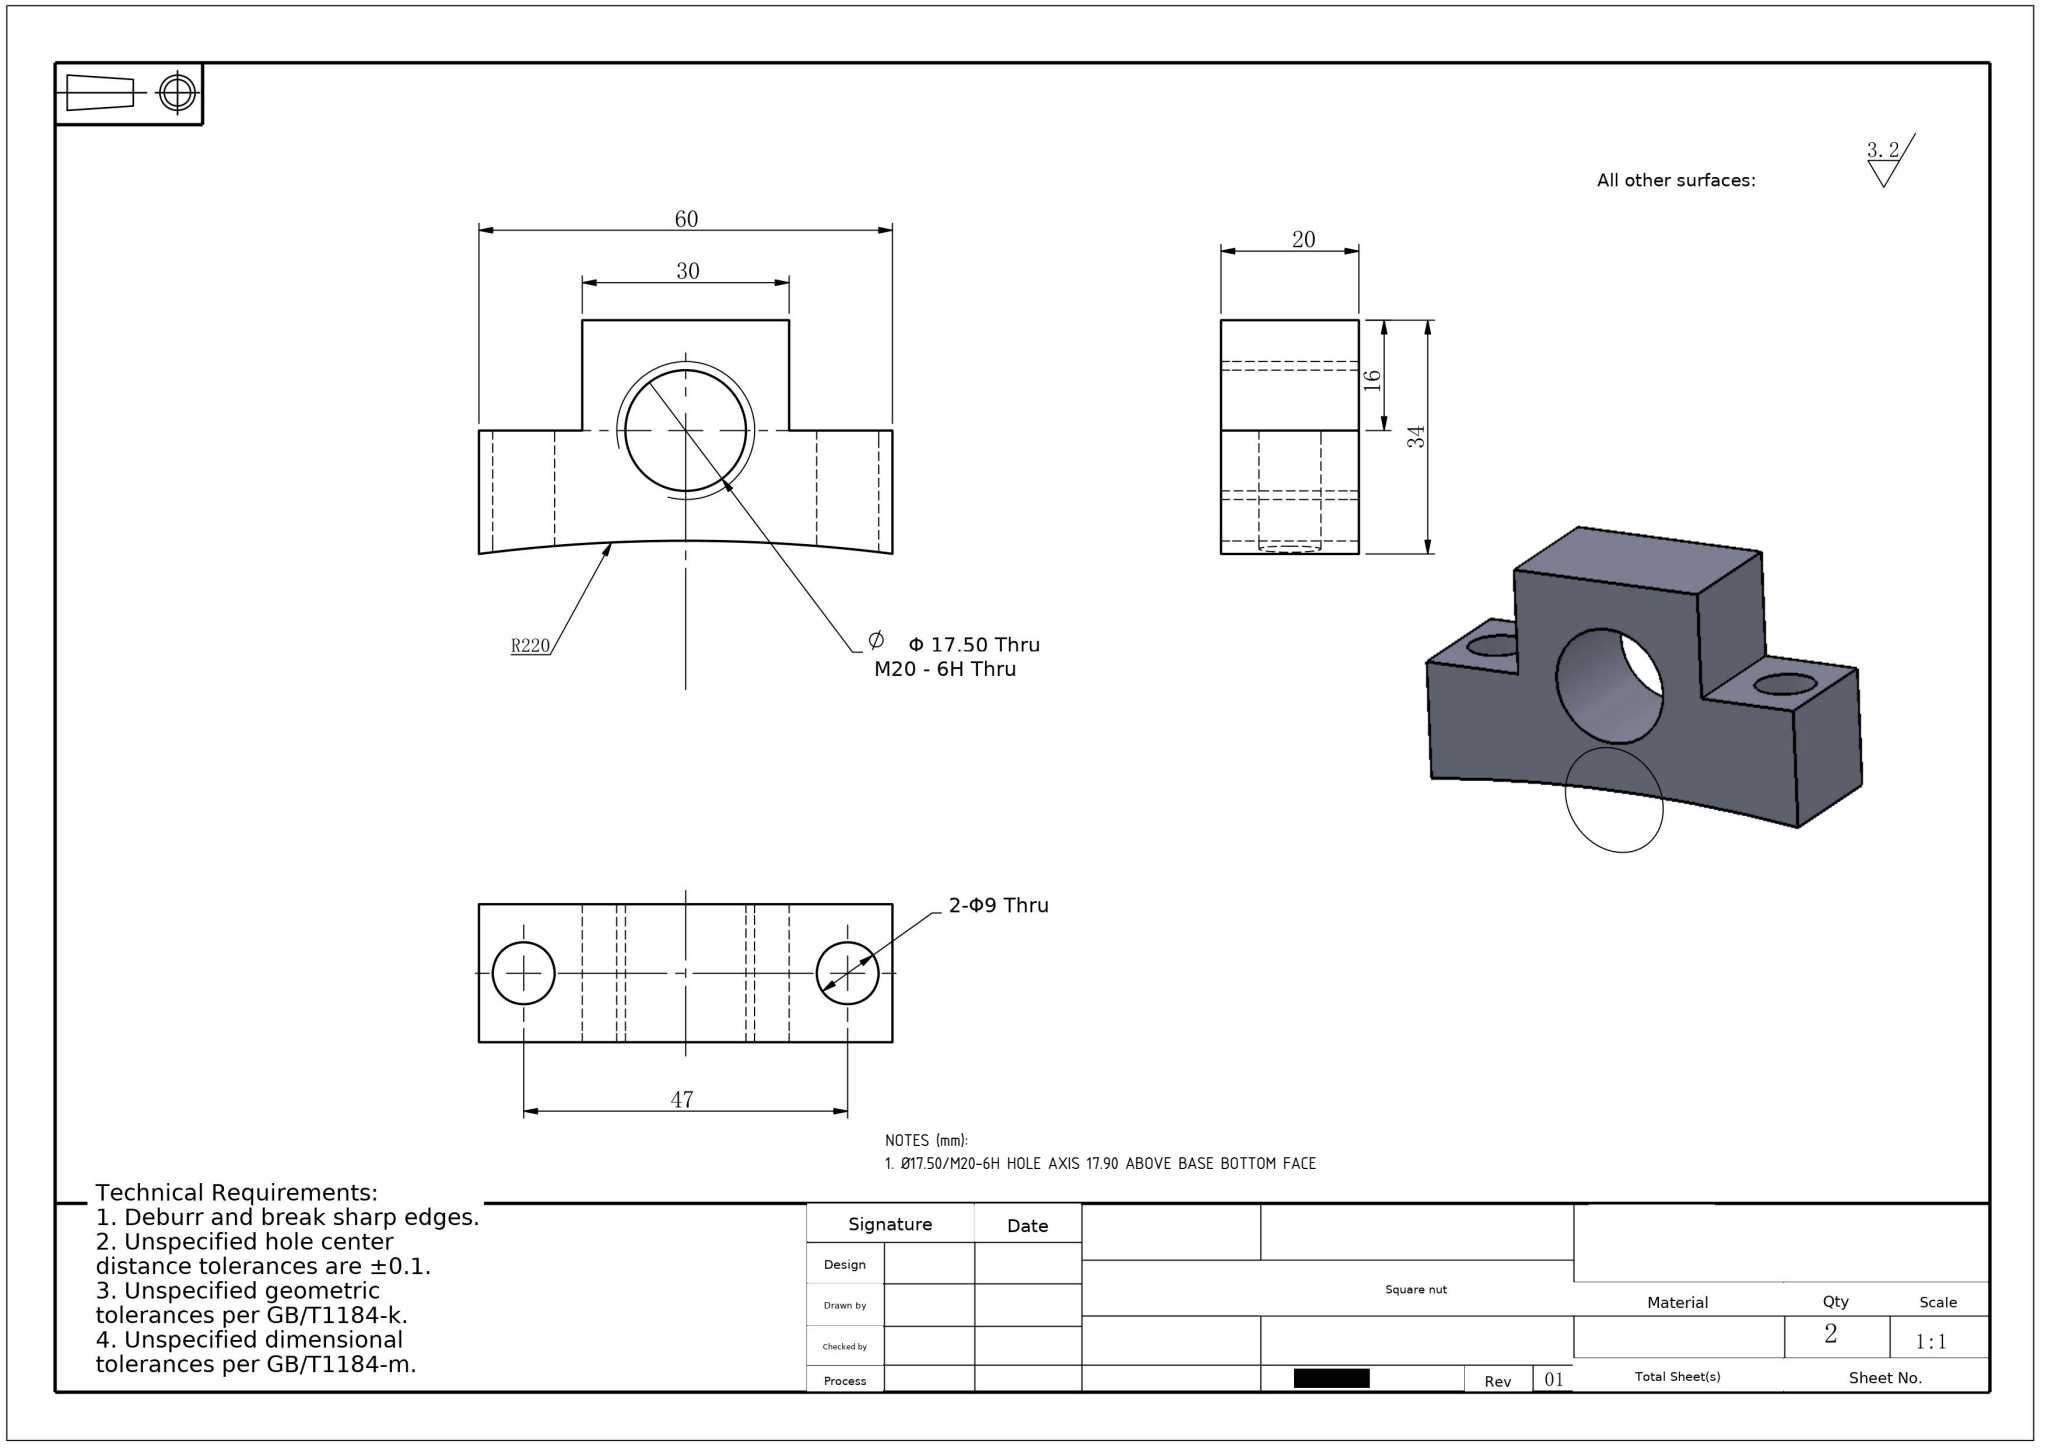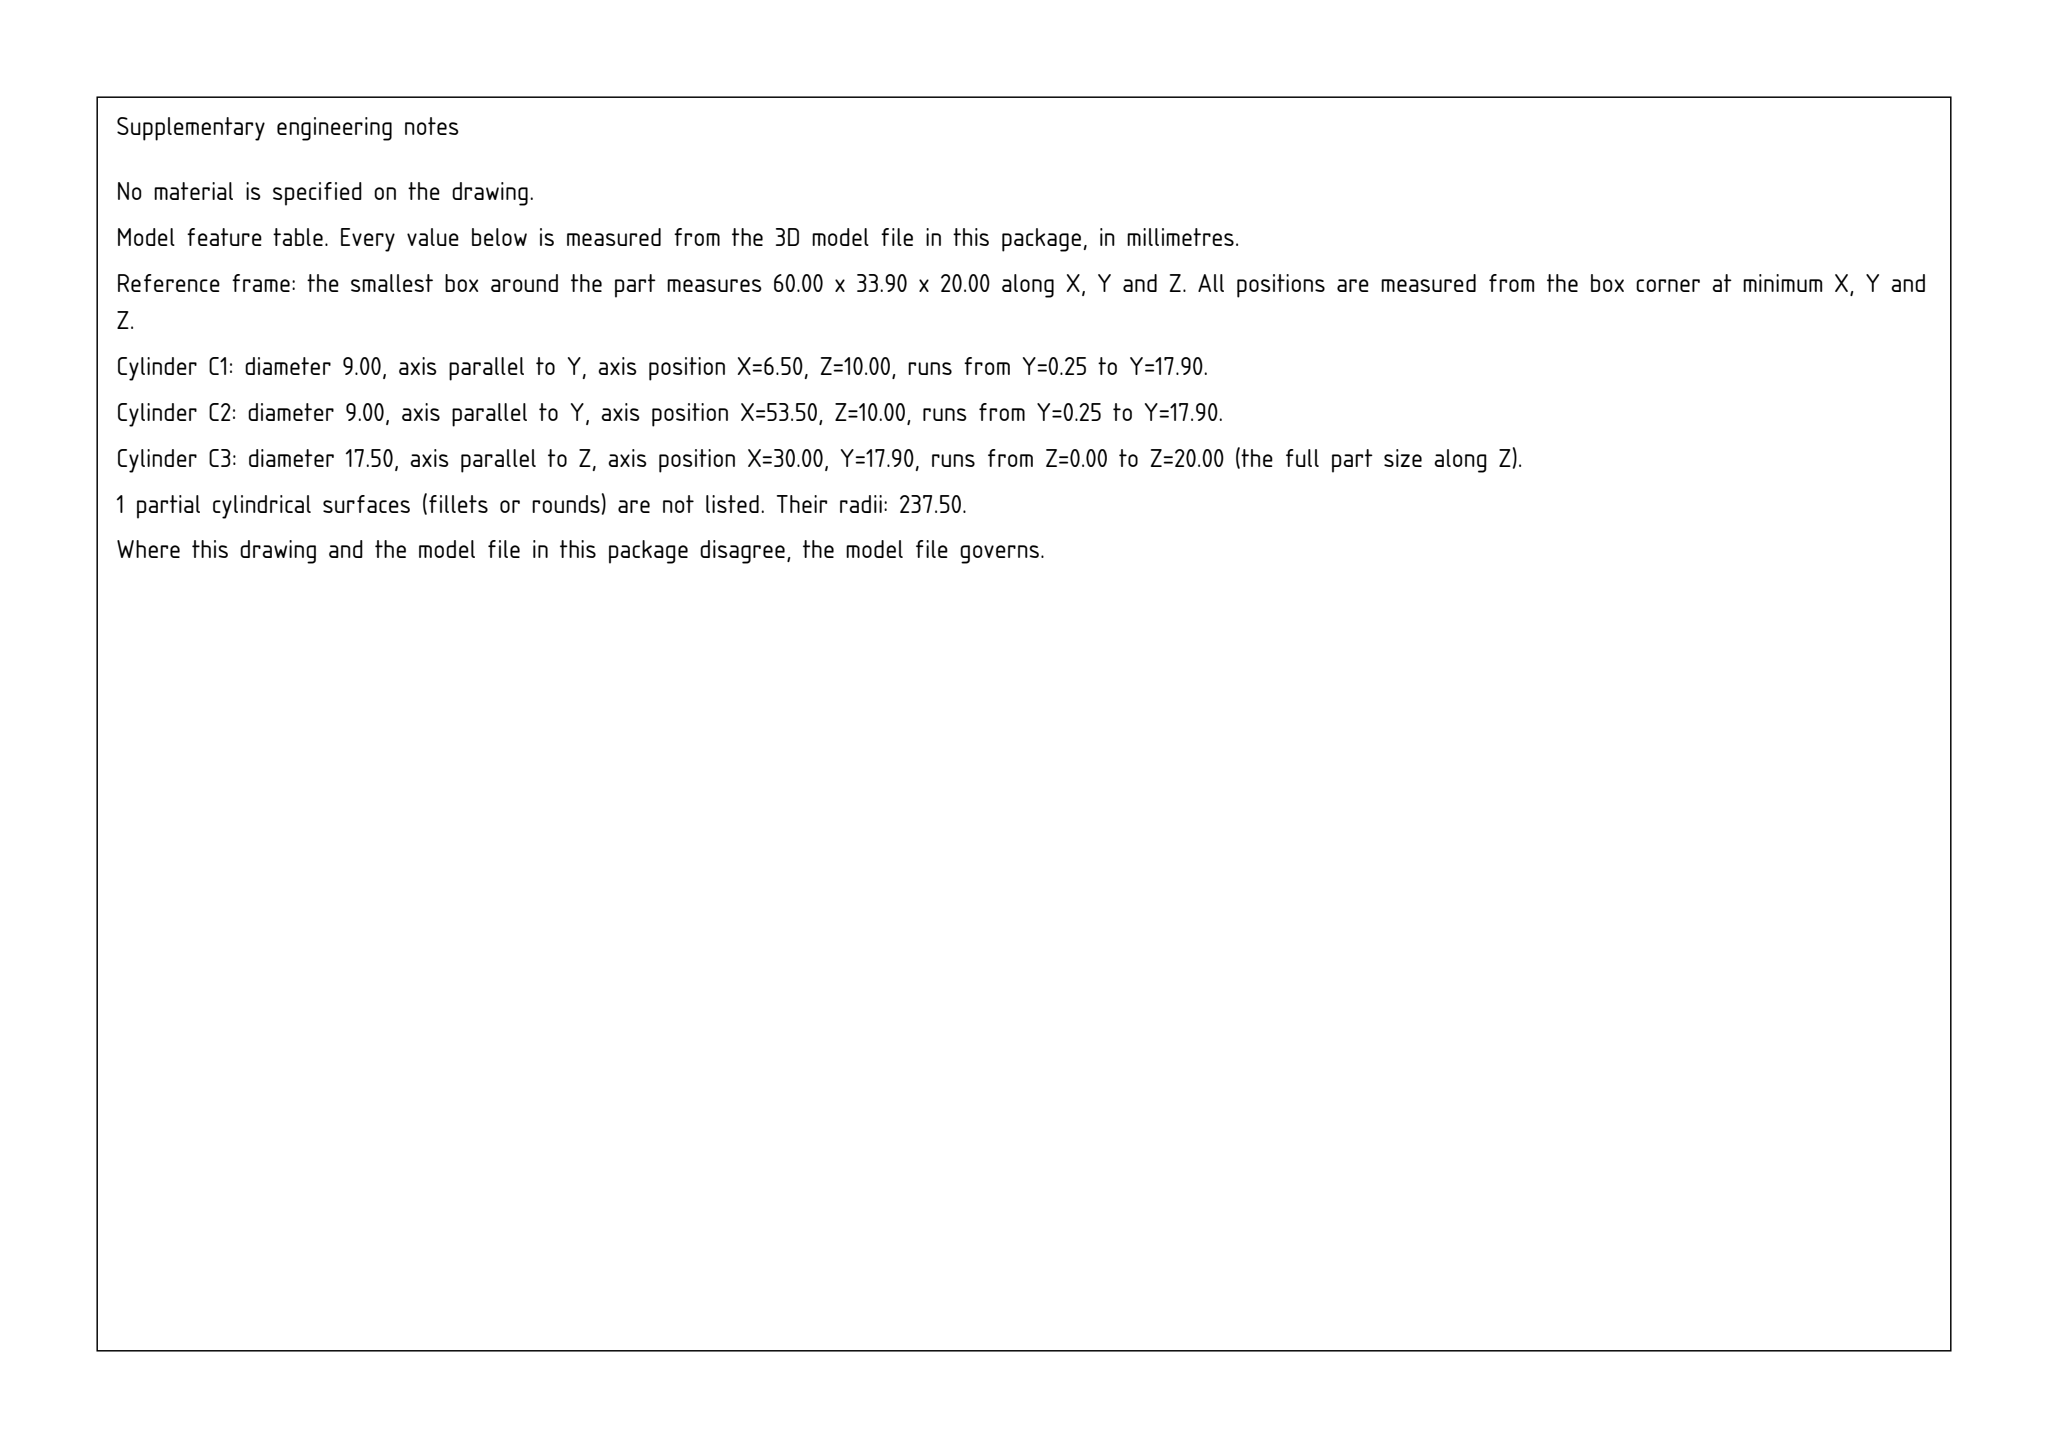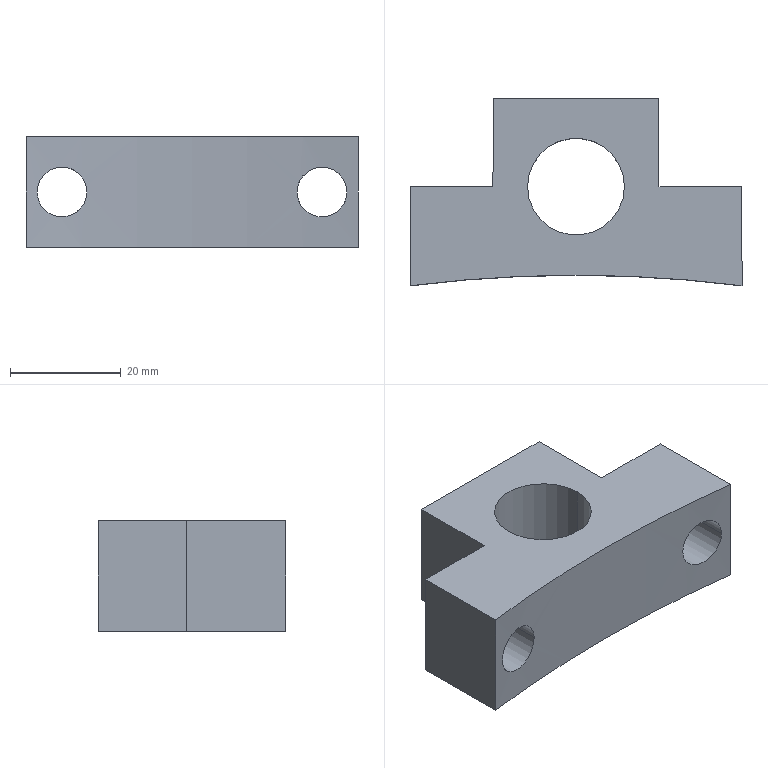Part | SolidWorks | mm | 1 solid | 16 faces | box 60 x 33.9 x 20 mm | volume 22564 mm3 | plane 9 | cylinder 7 | commonest cylinder face diameters 9 x4 17.5 x2 475 x1
Drawing notes:
Ø17.50/M20-6H HOLE AXIS 17.90 ABOVE BASE BOTTOM FACE | from the solid: cylinder [17.5,"z",[30.0,17.9,null],20.0] with bbox y=33.902 measured from min corner (bottom face)
build123d program:
from build123d import *

# Parameters (mm, degrees)
BOSS_EXTRUDE1_DEPTH = 20
M20_TAPPED_HOLE1_D  = 17.5
SKETCH4_R           = 4.5
CUT_EXTRUDE1_DEPTH  = 77.234


with BuildPart() as part:
    # Sketch1 → Boss-Extrude1 (new body)
    with BuildSketch(Plane.XY):
        with BuildLine():
            Line((-56.353, 59.764), (-26.353, 59.764))
            Line((-26.353, 59.764), (-26.353, 43.764))
            Line((-26.353, 43.764), (-11.353, 43.764))
            Line((-11.353, 43.764), (-11.353, 25.862))
            ThreePointArc((-11.353, 25.862), (-41.353, 27.764), (-71.353, 25.862))
            Line((-71.353, 25.862), (-71.353, 43.764))
            Line((-71.353, 43.764), (-56.353, 43.764))
            Line((-56.353, 43.764), (-56.353, 59.764))
        make_face()
    extrude(amount=BOSS_EXTRUDE1_DEPTH)

    # M20 Tapped Hole1 (through all)
    with Locations(Plane.XY.offset(20)):
        with Locations((-41.353, 43.764)):
            Hole(M20_TAPPED_HOLE1_D / 2)

    # Sketch4 → Cut-Extrude1 (cut, through all)
    with BuildSketch(Plane(origin=(0, 43.764, 0), x_dir=(-1, 0, 0), z_dir=(0, 1, 0))):
        with Locations((64.853, 10)):
            Circle(SKETCH4_R)
        with Locations((17.853, 10)):
            Circle(SKETCH4_R)
    extrude(amount=-CUT_EXTRUDE1_DEPTH, mode=Mode.SUBTRACT)


solid = part.part
STEP:
#1=CARTESIAN_POINT('',(-13.353,26.108,10.));
#2=VERTEX_POINT('',#1);
#3=CARTESIAN_POINT('',(-22.353,27.003,10.));
#4=VERTEX_POINT('',#3);
#5=CARTESIAN_POINT('',(-13.353,26.108,10.));
#6=CARTESIAN_POINT('',(-13.353,26.108,9.706));
#7=CARTESIAN_POINT('',(-13.381,26.112,9.413));
#8=CARTESIAN_POINT('',(-13.497,26.125,8.832));
#9=CARTESIAN_POINT('',(-13.584,26.135,8.547));
#10=CARTESIAN_POINT('',(-13.809,26.162,8.005));
#11=CARTESIAN_POINT('',(-13.948,26.178,7.743));
#12=CARTESIAN_POINT('',(-14.278,26.216,7.251));
#13=CARTESIAN_POINT('',(-14.464,26.238,7.024));
#14=CARTESIAN_POINT('',(-14.879,26.284,6.61));
#15=CARTESIAN_POINT('',(-15.11,26.31,6.42));
#16=CARTESIAN_POINT('',(-15.599,26.364,6.094));
#17=CARTESIAN_POINT('',(-15.857,26.392,5.956));
#18=CARTESIAN_POINT('',(-16.4,26.45,5.731));
#19=CARTESIAN_POINT('',(-16.685,26.48,5.644));
#20=CARTESIAN_POINT('',(-17.259,26.539,5.53));
#21=CARTESIAN_POINT('',(-17.55,26.569,5.5));
#22=CARTESIAN_POINT('',(-18.143,26.628,5.5));
#23=CARTESIAN_POINT('',(-18.435,26.656,5.528));
#24=CARTESIAN_POINT('',(-19.009,26.711,5.641));
#25=CARTESIAN_POINT('',(-19.294,26.738,5.727));
#26=CARTESIAN_POINT('',(-19.84,26.788,5.952));
#27=CARTESIAN_POINT('',(-20.098,26.812,6.089));
#28=CARTESIAN_POINT('',(-20.587,26.855,6.414));
#29=CARTESIAN_POINT('',(-20.819,26.875,6.604));
#30=CARTESIAN_POINT('',(-21.236,26.911,7.019));
#31=CARTESIAN_POINT('',(-21.423,26.927,7.245));
#32=CARTESIAN_POINT('',(-21.753,26.954,7.736));
#33=CARTESIAN_POINT('',(-21.894,26.966,7.999));
#34=CARTESIAN_POINT('',(-22.12,26.984,8.541));
#35=CARTESIAN_POINT('',(-22.206,26.991,8.823));
#36=CARTESIAN_POINT('',(-22.323,27.001,9.407));
#37=CARTESIAN_POINT('',(-22.353,27.003,9.702));
#38=CARTESIAN_POINT('',(-22.353,27.003,10.));
#39=B_SPLINE_CURVE_WITH_KNOTS('',3,(#5,#6,#7,#8,#9,#10,#11,#12,#13,#14,#15,#16,#17,#18,#19,#20,#21,#22,#23,#24,#25,#26,#27,#28,#29,#30,#31,#32,#33,#34,#35,#36,#37,#38),.UNSPECIFIED.,.F.,.F.,(4,2,2,2,2,2,2,2,2,2,2,2,2,2,2,2,4),(0.0141,0.01499,0.01587,0.01675,0.01763,0.01851,0.01939,0.02027,0.02116,0.02204,0.02292,0.0238,0.02468,0.02556,0.02644,0.02732,0.02821),.UNSPECIFIED.);
#40=EDGE_CURVE('',#2,#4,#39,.T.);
#41=ORIENTED_EDGE('',*,*,#40,.F.);
#42=CARTESIAN_POINT('',(-13.353,43.764,10.));
#43=VERTEX_POINT('',#42);
#44=CARTESIAN_POINT('',(-13.353,25.862,10.));
#45=DIRECTION('',(0.,1.,0.));
#46=VECTOR('',#45,1000.);
#47=LINE('',#44,#46);
#48=EDGE_CURVE('',#2,#43,#47,.T.);
#49=ORIENTED_EDGE('',*,*,#48,.T.);
#50=CARTESIAN_POINT('',(-22.353,43.764,10.));
#51=VERTEX_POINT('',#50);
#52=CARTESIAN_POINT('',(-17.853,43.764,10.));
#53=DIRECTION('',(0.,1.,0.));
#54=DIRECTION('',(1.,0.,0.));
#55=AXIS2_PLACEMENT_3D('',#52,#53,#54);
#56=CIRCLE('',#55,4.5);
#57=EDGE_CURVE('',#43,#51,#56,.T.);
#58=ORIENTED_EDGE('',*,*,#57,.T.);
#59=CARTESIAN_POINT('',(-22.353,25.862,10.));
#60=DIRECTION('',(0.,1.,0.));
#61=VECTOR('',#60,1000.);
#62=LINE('',#59,#61);
#63=EDGE_CURVE('',#4,#51,#62,.T.);
#64=ORIENTED_EDGE('',*,*,#63,.F.);
#65=EDGE_LOOP('',(#41,#49,#58,#64));
#66=FACE_OUTER_BOUND('',#65,.T.);
#67=CARTESIAN_POINT('',(-17.853,25.862,10.));
#68=DIRECTION('',(0.,1.,0.));
#69=DIRECTION('',(-1.,0.,0.));
#70=AXIS2_PLACEMENT_3D('',#67,#68,#69);
#71=CYLINDRICAL_SURFACE('',#70,4.5);
#72=ADVANCED_FACE('',(#66),#71,.F.);
#73=CARTESIAN_POINT('',(-60.353,27.003,10.));
#74=VERTEX_POINT('',#73);
#75=CARTESIAN_POINT('',(-69.353,26.108,10.));
#76=VERTEX_POINT('',#75);
#77=CARTESIAN_POINT('',(-60.353,27.003,10.));
#78=CARTESIAN_POINT('',(-60.353,27.003,9.706));
#79=CARTESIAN_POINT('',(-60.381,27.001,9.413));
#80=CARTESIAN_POINT('',(-60.497,26.992,8.832));
#81=CARTESIAN_POINT('',(-60.584,26.985,8.547));
#82=CARTESIAN_POINT('',(-60.809,26.966,8.004));
#83=CARTESIAN_POINT('',(-60.949,26.955,7.743));
#84=CARTESIAN_POINT('',(-61.279,26.927,7.25));
#85=CARTESIAN_POINT('',(-61.465,26.911,7.023));
#86=CARTESIAN_POINT('',(-61.881,26.876,6.608));
#87=CARTESIAN_POINT('',(-62.113,26.855,6.418));
#88=CARTESIAN_POINT('',(-62.602,26.812,6.092));
#89=CARTESIAN_POINT('',(-62.861,26.789,5.954));
#90=CARTESIAN_POINT('',(-63.405,26.739,5.729));
#91=CARTESIAN_POINT('',(-63.69,26.712,5.643));
#92=CARTESIAN_POINT('',(-64.265,26.657,5.529));
#93=CARTESIAN_POINT('',(-64.556,26.628,5.5));
#94=CARTESIAN_POINT('',(-65.148,26.57,5.5));
#95=CARTESIAN_POINT('',(-65.441,26.54,5.529));
#96=CARTESIAN_POINT('',(-66.014,26.481,5.643));
#97=CARTESIAN_POINT('',(-66.299,26.451,5.729));
#98=CARTESIAN_POINT('',(-66.843,26.393,5.954));
#99=CARTESIAN_POINT('',(-67.101,26.365,6.091));
#100=CARTESIAN_POINT('',(-67.59,26.311,6.416));
#101=CARTESIAN_POINT('',(-67.821,26.285,6.606));
#102=CARTESIAN_POINT('',(-68.237,26.238,7.02));
#103=CARTESIAN_POINT('',(-68.424,26.217,7.246));
#104=CARTESIAN_POINT('',(-68.753,26.179,7.736));
#105=CARTESIAN_POINT('',(-68.894,26.162,7.999));
#106=CARTESIAN_POINT('',(-69.12,26.136,8.541));
#107=CARTESIAN_POINT('',(-69.206,26.125,8.824));
#108=CARTESIAN_POINT('',(-69.323,26.112,9.407));
#109=CARTESIAN_POINT('',(-69.353,26.108,9.702));
#110=CARTESIAN_POINT('',(-69.353,26.108,10.));
#111=B_SPLINE_CURVE_WITH_KNOTS('',3,(#77,#78,#79,#80,#81,#82,#83,#84,#85,#86,#87,#88,#89,#90,#91,#92,#93,#94,#95,#96,#97,#98,#99,#100,#101,#102,#103,#104,#105,#106,#107,#108,#109,#110),.UNSPECIFIED.,.F.,.F.,(4,2,2,2,2,2,2,2,2,2,2,2,2,2,2,2,4),(0.0141,0.01499,0.01587,0.01675,0.01763,0.01851,0.01939,0.02027,0.02116,0.02204,0.02292,0.0238,0.02468,0.02556,0.02644,0.02732,0.02821),.UNSPECIFIED.);
#112=EDGE_CURVE('',#74,#76,#111,.T.);
#113=ORIENTED_EDGE('',*,*,#112,.F.);
#114=CARTESIAN_POINT('',(-60.353,43.764,10.));
#115=VERTEX_POINT('',#114);
#116=CARTESIAN_POINT('',(-60.353,25.862,10.));
#117=DIRECTION('',(0.,1.,0.));
#118=VECTOR('',#117,1000.);
#119=LINE('',#116,#118);
#120=EDGE_CURVE('',#74,#115,#119,.T.);
#121=ORIENTED_EDGE('',*,*,#120,.T.);
#122=CARTESIAN_POINT('',(-69.353,43.764,10.));
#123=VERTEX_POINT('',#122);
#124=CARTESIAN_POINT('',(-64.853,43.764,10.));
#125=DIRECTION('',(0.,1.,0.));
#126=DIRECTION('',(-1.,0.,0.));
#127=AXIS2_PLACEMENT_3D('',#124,#125,#126);
#128=CIRCLE('',#127,4.5);
#129=EDGE_CURVE('',#115,#123,#128,.T.);
#130=ORIENTED_EDGE('',*,*,#129,.T.);
#131=CARTESIAN_POINT('',(-69.353,25.862,10.));
#132=DIRECTION('',(0.,1.,0.));
#133=VECTOR('',#132,1000.);
#134=LINE('',#131,#133);
#135=EDGE_CURVE('',#76,#123,#134,.T.);
#136=ORIENTED_EDGE('',*,*,#135,.F.);
#137=EDGE_LOOP('',(#113,#121,#130,#136));
#138=FACE_OUTER_BOUND('',#137,.T.);
#139=CARTESIAN_POINT('',(-64.853,25.862,10.));
#140=DIRECTION('',(0.,1.,0.));
#141=DIRECTION('',(-1.,0.,0.));
#142=AXIS2_PLACEMENT_3D('',#139,#140,#141);
#143=CYLINDRICAL_SURFACE('',#142,4.5);
#144=ADVANCED_FACE('',(#138),#143,.F.);
#145=CARTESIAN_POINT('',(-50.103,43.764,0.));
#146=VERTEX_POINT('',#145);
#147=CARTESIAN_POINT('',(-32.603,43.764,0.));
#148=VERTEX_POINT('',#147);
#149=CARTESIAN_POINT('',(-41.353,43.764,0.));
#150=DIRECTION('',(0.,0.,1.));
#151=DIRECTION('',(1.,0.,0.));
#152=AXIS2_PLACEMENT_3D('',#149,#150,#151);
#153=CIRCLE('',#152,8.75);
#154=EDGE_CURVE('',#146,#148,#153,.T.);
#155=ORIENTED_EDGE('',*,*,#154,.F.);
#156=CARTESIAN_POINT('',(-50.103,43.764,20.));
#157=VERTEX_POINT('',#156);
#158=CARTESIAN_POINT('',(-50.103,43.764,20.));
#159=DIRECTION('',(0.,0.,1.));
#160=VECTOR('',#159,1000.);
#161=LINE('',#158,#160);
#162=EDGE_CURVE('',#146,#157,#161,.T.);
#163=ORIENTED_EDGE('',*,*,#162,.T.);
#164=CARTESIAN_POINT('',(-32.603,43.764,20.));
#165=VERTEX_POINT('',#164);
#166=CARTESIAN_POINT('',(-41.353,43.764,20.));
#167=DIRECTION('',(0.,0.,1.));
#168=DIRECTION('',(1.,0.,0.));
#169=AXIS2_PLACEMENT_3D('',#166,#167,#168);
#170=CIRCLE('',#169,8.75);
#171=EDGE_CURVE('',#157,#165,#170,.T.);
#172=ORIENTED_EDGE('',*,*,#171,.T.);
#173=CARTESIAN_POINT('',(-32.603,43.764,20.));
#174=DIRECTION('',(0.,0.,1.));
#175=VECTOR('',#174,1000.);
#176=LINE('',#173,#175);
#177=EDGE_CURVE('',#148,#165,#176,.T.);
#178=ORIENTED_EDGE('',*,*,#177,.F.);
#179=EDGE_LOOP('',(#155,#163,#172,#178));
#180=FACE_OUTER_BOUND('',#179,.T.);
#181=CARTESIAN_POINT('',(-41.353,43.764,20.));
#182=DIRECTION('',(0.,0.,1.));
#183=DIRECTION('',(1.,0.,0.));
#184=AXIS2_PLACEMENT_3D('',#181,#182,#183);
#185=CYLINDRICAL_SURFACE('',#184,8.75);
#186=ADVANCED_FACE('',(#180),#185,.F.);
#187=CARTESIAN_POINT('',(-56.353,59.764,0.));
#188=VERTEX_POINT('',#187);
#189=CARTESIAN_POINT('',(-56.353,43.764,0.));
#190=VERTEX_POINT('',#189);
#191=CARTESIAN_POINT('',(-56.353,59.764,0.));
#192=DIRECTION('',(-0.,-1.,0.));
#193=VECTOR('',#192,1000.);
#194=LINE('',#191,#193);
#195=EDGE_CURVE('',#188,#190,#194,.T.);
#196=ORIENTED_EDGE('',*,*,#195,.T.);
#197=CARTESIAN_POINT('',(-56.353,43.764,20.));
#198=VERTEX_POINT('',#197);
#199=CARTESIAN_POINT('',(-56.353,43.764,20.));
#200=DIRECTION('',(0.,0.,-1.));
#201=VECTOR('',#200,1000.);
#202=LINE('',#199,#201);
#203=EDGE_CURVE('',#198,#190,#202,.T.);
#204=ORIENTED_EDGE('',*,*,#203,.F.);
#205=CARTESIAN_POINT('',(-56.353,59.764,20.));
#206=VERTEX_POINT('',#205);
#207=CARTESIAN_POINT('',(-56.353,59.764,20.));
#208=DIRECTION('',(-0.,-1.,0.));
#209=VECTOR('',#208,1000.);
#210=LINE('',#207,#209);
#211=EDGE_CURVE('',#206,#198,#210,.T.);
#212=ORIENTED_EDGE('',*,*,#211,.F.);
#213=CARTESIAN_POINT('',(-56.353,59.764,20.));
#214=DIRECTION('',(0.,0.,-1.));
#215=VECTOR('',#214,1000.);
#216=LINE('',#213,#215);
#217=EDGE_CURVE('',#206,#188,#216,.T.);
#218=ORIENTED_EDGE('',*,*,#217,.T.);
#219=EDGE_LOOP('',(#196,#204,#212,#218));
#220=FACE_OUTER_BOUND('',#219,.T.);
#221=CARTESIAN_POINT('',(-56.353,59.764,20.));
#222=DIRECTION('',(1.,-0.,0.));
#223=DIRECTION('',(0.,1.,0.));
#224=AXIS2_PLACEMENT_3D('',#221,#222,#223);
#225=PLANE('',#224);
#226=ADVANCED_FACE('',(#220),#225,.F.);
#227=CARTESIAN_POINT('',(-64.853,43.764,10.));
#228=DIRECTION('',(0.,1.,0.));
#229=DIRECTION('',(-1.,0.,0.));
#230=AXIS2_PLACEMENT_3D('',#227,#228,#229);
#231=CIRCLE('',#230,4.5);
#232=EDGE_CURVE('',#123,#115,#231,.T.);
#233=ORIENTED_EDGE('',*,*,#232,.F.);
#234=ORIENTED_EDGE('',*,*,#129,.F.);
#235=EDGE_LOOP('',(#233,#234));
#236=FACE_BOUND('',#235,.T.);
#237=CARTESIAN_POINT('',(-71.353,43.764,0.));
#238=VERTEX_POINT('',#237);
#239=CARTESIAN_POINT('',(-71.353,43.764,0.));
#240=DIRECTION('',(-1.,0.,0.));
#241=VECTOR('',#240,1000.);
#242=LINE('',#239,#241);
#243=EDGE_CURVE('',#190,#238,#242,.T.);
#244=ORIENTED_EDGE('',*,*,#243,.T.);
#245=CARTESIAN_POINT('',(-71.353,43.764,20.));
#246=VERTEX_POINT('',#245);
#247=CARTESIAN_POINT('',(-71.353,43.764,20.));
#248=DIRECTION('',(0.,0.,-1.));
#249=VECTOR('',#248,1000.);
#250=LINE('',#247,#249);
#251=EDGE_CURVE('',#246,#238,#250,.T.);
#252=ORIENTED_EDGE('',*,*,#251,.F.);
#253=CARTESIAN_POINT('',(-71.353,43.764,20.));
#254=DIRECTION('',(-1.,0.,0.));
#255=VECTOR('',#254,1000.);
#256=LINE('',#253,#255);
#257=EDGE_CURVE('',#198,#246,#256,.T.);
#258=ORIENTED_EDGE('',*,*,#257,.F.);
#259=ORIENTED_EDGE('',*,*,#203,.T.);
#260=EDGE_LOOP('',(#244,#252,#258,#259));
#261=FACE_OUTER_BOUND('',#260,.T.);
#262=CARTESIAN_POINT('',(-71.353,43.764,20.));
#263=DIRECTION('',(0.,-1.,0.));
#264=DIRECTION('',(0.,0.,-1.));
#265=AXIS2_PLACEMENT_3D('',#262,#263,#264);
#266=PLANE('',#265);
#267=ADVANCED_FACE('',(#236,#261),#266,.F.);
#268=CARTESIAN_POINT('',(-71.353,25.862,0.));
#269=VERTEX_POINT('',#268);
#270=CARTESIAN_POINT('',(-71.353,43.764,0.));
#271=DIRECTION('',(-0.,-1.,0.));
#272=VECTOR('',#271,1000.);
#273=LINE('',#270,#272);
#274=EDGE_CURVE('',#238,#269,#273,.T.);
#275=ORIENTED_EDGE('',*,*,#274,.T.);
#276=CARTESIAN_POINT('',(-71.353,25.862,20.));
#277=VERTEX_POINT('',#276);
#278=CARTESIAN_POINT('',(-71.353,25.862,20.));
#279=DIRECTION('',(0.,0.,-1.));
#280=VECTOR('',#279,1000.);
#281=LINE('',#278,#280);
#282=EDGE_CURVE('',#277,#269,#281,.T.);
#283=ORIENTED_EDGE('',*,*,#282,.F.);
#284=CARTESIAN_POINT('',(-71.353,43.764,20.));
#285=DIRECTION('',(-0.,-1.,0.));
#286=VECTOR('',#285,1000.);
#287=LINE('',#284,#286);
#288=EDGE_CURVE('',#246,#277,#287,.T.);
#289=ORIENTED_EDGE('',*,*,#288,.F.);
#290=ORIENTED_EDGE('',*,*,#251,.T.);
#291=EDGE_LOOP('',(#275,#283,#289,#290));
#292=FACE_OUTER_BOUND('',#291,.T.);
#293=CARTESIAN_POINT('',(-71.353,43.764,20.));
#294=DIRECTION('',(1.,-0.,0.));
#295=DIRECTION('',(0.,1.,0.));
#296=AXIS2_PLACEMENT_3D('',#293,#294,#295);
#297=PLANE('',#296);
#298=ADVANCED_FACE('',(#292),#297,.F.);
#299=CARTESIAN_POINT('',(-22.353,27.003,10.));
#300=CARTESIAN_POINT('',(-22.353,27.003,10.298));
#301=CARTESIAN_POINT('',(-22.323,27.001,10.591));
#302=CARTESIAN_POINT('',(-22.208,26.992,11.168));
#303=CARTESIAN_POINT('',(-22.121,26.985,11.454));
#304=CARTESIAN_POINT('',(-21.895,26.966,12.));
#305=CARTESIAN_POINT('',(-21.756,26.955,12.259));
#306=CARTESIAN_POINT('',(-21.428,26.927,12.748));
#307=CARTESIAN_POINT('',(-21.237,26.911,12.98));
#308=CARTESIAN_POINT('',(-20.821,26.875,13.395));
#309=CARTESIAN_POINT('',(-20.594,26.856,13.581));
#310=CARTESIAN_POINT('',(-20.101,26.812,13.909));
#311=CARTESIAN_POINT('',(-19.84,26.788,14.048));
#312=CARTESIAN_POINT('',(-19.299,26.738,14.271));
#313=CARTESIAN_POINT('',(-19.015,26.712,14.357));
#314=CARTESIAN_POINT('',(-18.435,26.656,14.472));
#315=CARTESIAN_POINT('',(-18.144,26.628,14.5));
#316=CARTESIAN_POINT('',(-17.558,26.57,14.5));
#317=CARTESIAN_POINT('',(-17.261,26.54,14.471));
#318=CARTESIAN_POINT('',(-16.685,26.48,14.356));
#319=CARTESIAN_POINT('',(-16.406,26.451,14.271));
#320=CARTESIAN_POINT('',(-15.862,26.393,14.046));
#321=CARTESIAN_POINT('',(-15.599,26.364,13.906));
#322=CARTESIAN_POINT('',(-15.112,26.31,13.581));
#323=CARTESIAN_POINT('',(-14.885,26.285,13.395));
#324=CARTESIAN_POINT('',(-14.464,26.238,12.976));
#325=CARTESIAN_POINT('',(-14.278,26.216,12.749));
#326=CARTESIAN_POINT('',(-13.951,26.178,12.261));
#327=CARTESIAN_POINT('',(-13.81,26.162,11.998));
#328=CARTESIAN_POINT('',(-13.583,26.135,11.452));
#329=CARTESIAN_POINT('',(-13.498,26.125,11.171));
#330=CARTESIAN_POINT('',(-13.382,26.112,10.594));
#331=CARTESIAN_POINT('',(-13.353,26.108,10.294));
#332=CARTESIAN_POINT('',(-13.353,26.108,10.));
#333=B_SPLINE_CURVE_WITH_KNOTS('',3,(#299,#300,#301,#302,#303,#304,#305,#306,#307,#308,#309,#310,#311,#312,#313,#314,#315,#316,#317,#318,#319,#320,#321,#322,#323,#324,#325,#326,#327,#328,#329,#330,#331,#332),.UNSPECIFIED.,.F.,.F.,(4,2,2,2,2,2,2,2,2,2,2,2,2,2,2,2,4),(0.,0.0008815,0.001763,0.002645,0.003526,0.004408,0.005289,0.006171,0.007052,0.007934,0.008815,0.009697,0.01058,0.01146,0.01234,0.01322,0.0141),.UNSPECIFIED.);
#334=EDGE_CURVE('',#4,#2,#333,.T.);
#335=ORIENTED_EDGE('',*,*,#334,.T.);
#336=ORIENTED_EDGE('',*,*,#40,.T.);
#337=EDGE_LOOP('',(#335,#336));
#338=FACE_BOUND('',#337,.T.);
#339=CARTESIAN_POINT('',(-69.353,26.108,10.));
#340=CARTESIAN_POINT('',(-69.353,26.108,10.298));
#341=CARTESIAN_POINT('',(-69.323,26.112,10.591));
#342=CARTESIAN_POINT('',(-69.208,26.125,11.168));
#343=CARTESIAN_POINT('',(-69.121,26.135,11.454));
#344=CARTESIAN_POINT('',(-68.895,26.162,12.));
#345=CARTESIAN_POINT('',(-68.756,26.178,12.258));
#346=CARTESIAN_POINT('',(-68.429,26.216,12.747));
#347=CARTESIAN_POINT('',(-68.238,26.238,12.979));
#348=CARTESIAN_POINT('',(-67.823,26.285,13.393));
#349=CARTESIAN_POINT('',(-67.596,26.31,13.579));
#350=CARTESIAN_POINT('',(-67.105,26.364,13.907));
#351=CARTESIAN_POINT('',(-66.843,26.393,14.046));
#352=CARTESIAN_POINT('',(-66.303,26.45,14.27));
#353=CARTESIAN_POINT('',(-66.02,26.48,14.356));
#354=CARTESIAN_POINT('',(-65.441,26.54,14.471));
#355=CARTESIAN_POINT('',(-65.15,26.569,14.5));
#356=CARTESIAN_POINT('',(-64.564,26.628,14.5));
#357=CARTESIAN_POINT('',(-64.266,26.657,14.471));
#358=CARTESIAN_POINT('',(-63.69,26.712,14.357));
#359=CARTESIAN_POINT('',(-63.41,26.738,14.273));
#360=CARTESIAN_POINT('',(-62.866,26.788,14.048));
#361=CARTESIAN_POINT('',(-62.602,26.812,13.908));
#362=CARTESIAN_POINT('',(-62.114,26.855,13.583));
#363=CARTESIAN_POINT('',(-61.887,26.875,13.397));
#364=CARTESIAN_POINT('',(-61.466,26.911,12.978));
#365=CARTESIAN_POINT('',(-61.278,26.927,12.75));
#366=CARTESIAN_POINT('',(-60.951,26.954,12.262));
#367=CARTESIAN_POINT('',(-60.81,26.966,11.999));
#368=CARTESIAN_POINT('',(-60.583,26.985,11.452));
#369=CARTESIAN_POINT('',(-60.498,26.992,11.171));
#370=CARTESIAN_POINT('',(-60.382,27.001,10.593));
#371=CARTESIAN_POINT('',(-60.353,27.003,10.294));
#372=CARTESIAN_POINT('',(-60.353,27.003,10.));
#373=B_SPLINE_CURVE_WITH_KNOTS('',3,(#339,#340,#341,#342,#343,#344,#345,#346,#347,#348,#349,#350,#351,#352,#353,#354,#355,#356,#357,#358,#359,#360,#361,#362,#363,#364,#365,#366,#367,#368,#369,#370,#371,#372),.UNSPECIFIED.,.F.,.F.,(4,2,2,2,2,2,2,2,2,2,2,2,2,2,2,2,4),(0.,0.0008815,0.001763,0.002645,0.003526,0.004408,0.005289,0.006171,0.007052,0.007934,0.008815,0.009697,0.01058,0.01146,0.01234,0.01322,0.0141),.UNSPECIFIED.);
#374=EDGE_CURVE('',#76,#74,#373,.T.);
#375=ORIENTED_EDGE('',*,*,#374,.T.);
#376=ORIENTED_EDGE('',*,*,#112,.T.);
#377=EDGE_LOOP('',(#375,#376));
#378=FACE_BOUND('',#377,.T.);
#379=CARTESIAN_POINT('',(-11.353,25.862,0.));
#380=VERTEX_POINT('',#379);
#381=CARTESIAN_POINT('',(-41.353,-209.736,0.));
#382=DIRECTION('',(0.,0.,-1.));
#383=DIRECTION('',(1.,0.,0.));
#384=AXIS2_PLACEMENT_3D('',#381,#382,#383);
#385=CIRCLE('',#384,237.5);
#386=EDGE_CURVE('',#269,#380,#385,.T.);
#387=ORIENTED_EDGE('',*,*,#386,.T.);
#388=CARTESIAN_POINT('',(-11.353,25.862,20.));
#389=VERTEX_POINT('',#388);
#390=CARTESIAN_POINT('',(-11.353,25.862,20.));
#391=DIRECTION('',(0.,0.,-1.));
#392=VECTOR('',#391,1000.);
#393=LINE('',#390,#392);
#394=EDGE_CURVE('',#389,#380,#393,.T.);
#395=ORIENTED_EDGE('',*,*,#394,.F.);
#396=CARTESIAN_POINT('',(-41.353,-209.736,20.));
#397=DIRECTION('',(0.,0.,-1.));
#398=DIRECTION('',(1.,0.,0.));
#399=AXIS2_PLACEMENT_3D('',#396,#397,#398);
#400=CIRCLE('',#399,237.5);
#401=EDGE_CURVE('',#277,#389,#400,.T.);
#402=ORIENTED_EDGE('',*,*,#401,.F.);
#403=ORIENTED_EDGE('',*,*,#282,.T.);
#404=EDGE_LOOP('',(#387,#395,#402,#403));
#405=FACE_OUTER_BOUND('',#404,.T.);
#406=CARTESIAN_POINT('',(-41.353,-209.736,20.));
#407=DIRECTION('',(0.,0.,-1.));
#408=DIRECTION('',(-1.,0.,0.));
#409=AXIS2_PLACEMENT_3D('',#406,#407,#408);
#410=CYLINDRICAL_SURFACE('',#409,237.5);
#411=ADVANCED_FACE('',(#338,#378,#405),#410,.F.);
#412=CARTESIAN_POINT('',(-11.353,43.764,0.));
#413=VERTEX_POINT('',#412);
#414=CARTESIAN_POINT('',(-11.353,43.764,0.));
#415=DIRECTION('',(-0.,1.,0.));
#416=VECTOR('',#415,1000.);
#417=LINE('',#414,#416);
#418=EDGE_CURVE('',#380,#413,#417,.T.);
#419=ORIENTED_EDGE('',*,*,#418,.T.);
#420=CARTESIAN_POINT('',(-11.353,43.764,20.));
#421=VERTEX_POINT('',#420);
#422=CARTESIAN_POINT('',(-11.353,43.764,20.));
#423=DIRECTION('',(0.,0.,-1.));
#424=VECTOR('',#423,1000.);
#425=LINE('',#422,#424);
#426=EDGE_CURVE('',#421,#413,#425,.T.);
#427=ORIENTED_EDGE('',*,*,#426,.F.);
#428=CARTESIAN_POINT('',(-11.353,43.764,20.));
#429=DIRECTION('',(-0.,1.,0.));
#430=VECTOR('',#429,1000.);
#431=LINE('',#428,#430);
#432=EDGE_CURVE('',#389,#421,#431,.T.);
#433=ORIENTED_EDGE('',*,*,#432,.F.);
#434=ORIENTED_EDGE('',*,*,#394,.T.);
#435=EDGE_LOOP('',(#419,#427,#433,#434));
#436=FACE_OUTER_BOUND('',#435,.T.);
#437=CARTESIAN_POINT('',(-11.353,43.764,20.));
#438=DIRECTION('',(-1.,-0.,0.));
#439=DIRECTION('',(0.,-1.,0.));
#440=AXIS2_PLACEMENT_3D('',#437,#438,#439);
#441=PLANE('',#440);
#442=ADVANCED_FACE('',(#436),#441,.F.);
#443=CARTESIAN_POINT('',(-17.853,43.764,10.));
#444=DIRECTION('',(0.,1.,0.));
#445=DIRECTION('',(1.,0.,0.));
#446=AXIS2_PLACEMENT_3D('',#443,#444,#445);
#447=CIRCLE('',#446,4.5);
#448=EDGE_CURVE('',#51,#43,#447,.T.);
#449=ORIENTED_EDGE('',*,*,#448,.F.);
#450=ORIENTED_EDGE('',*,*,#57,.F.);
#451=EDGE_LOOP('',(#449,#450));
#452=FACE_BOUND('',#451,.T.);
#453=CARTESIAN_POINT('',(-26.353,43.764,0.));
#454=VERTEX_POINT('',#453);
#455=CARTESIAN_POINT('',(-26.353,43.764,0.));
#456=DIRECTION('',(-1.,0.,0.));
#457=VECTOR('',#456,1000.);
#458=LINE('',#455,#457);
#459=EDGE_CURVE('',#413,#454,#458,.T.);
#460=ORIENTED_EDGE('',*,*,#459,.T.);
#461=CARTESIAN_POINT('',(-26.353,43.764,20.));
#462=VERTEX_POINT('',#461);
#463=CARTESIAN_POINT('',(-26.353,43.764,20.));
#464=DIRECTION('',(0.,0.,-1.));
#465=VECTOR('',#464,1000.);
#466=LINE('',#463,#465);
#467=EDGE_CURVE('',#462,#454,#466,.T.);
#468=ORIENTED_EDGE('',*,*,#467,.F.);
#469=CARTESIAN_POINT('',(-26.353,43.764,20.));
#470=DIRECTION('',(-1.,0.,0.));
#471=VECTOR('',#470,1000.);
#472=LINE('',#469,#471);
#473=EDGE_CURVE('',#421,#462,#472,.T.);
#474=ORIENTED_EDGE('',*,*,#473,.F.);
#475=ORIENTED_EDGE('',*,*,#426,.T.);
#476=EDGE_LOOP('',(#460,#468,#474,#475));
#477=FACE_OUTER_BOUND('',#476,.T.);
#478=CARTESIAN_POINT('',(-26.353,43.764,20.));
#479=DIRECTION('',(0.,-1.,0.));
#480=DIRECTION('',(0.,0.,-1.));
#481=AXIS2_PLACEMENT_3D('',#478,#479,#480);
#482=PLANE('',#481);
#483=ADVANCED_FACE('',(#452,#477),#482,.F.);
#484=CARTESIAN_POINT('',(-26.353,59.764,0.));
#485=VERTEX_POINT('',#484);
#486=CARTESIAN_POINT('',(-26.353,59.764,0.));
#487=DIRECTION('',(-0.,1.,0.));
#488=VECTOR('',#487,1000.);
#489=LINE('',#486,#488);
#490=EDGE_CURVE('',#454,#485,#489,.T.);
#491=ORIENTED_EDGE('',*,*,#490,.T.);
#492=CARTESIAN_POINT('',(-26.353,59.764,20.));
#493=VERTEX_POINT('',#492);
#494=CARTESIAN_POINT('',(-26.353,59.764,20.));
#495=DIRECTION('',(0.,0.,-1.));
#496=VECTOR('',#495,1000.);
#497=LINE('',#494,#496);
#498=EDGE_CURVE('',#493,#485,#497,.T.);
#499=ORIENTED_EDGE('',*,*,#498,.F.);
#500=CARTESIAN_POINT('',(-26.353,59.764,20.));
#501=DIRECTION('',(-0.,1.,0.));
#502=VECTOR('',#501,1000.);
#503=LINE('',#500,#502);
#504=EDGE_CURVE('',#462,#493,#503,.T.);
#505=ORIENTED_EDGE('',*,*,#504,.F.);
#506=ORIENTED_EDGE('',*,*,#467,.T.);
#507=EDGE_LOOP('',(#491,#499,#505,#506));
#508=FACE_OUTER_BOUND('',#507,.T.);
#509=CARTESIAN_POINT('',(-26.353,59.764,20.));
#510=DIRECTION('',(-1.,-0.,0.));
#511=DIRECTION('',(0.,-1.,0.));
#512=AXIS2_PLACEMENT_3D('',#509,#510,#511);
#513=PLANE('',#512);
#514=ADVANCED_FACE('',(#508),#513,.F.);
#515=CARTESIAN_POINT('',(-56.353,59.764,0.));
#516=DIRECTION('',(-1.,-0.,0.));
#517=VECTOR('',#516,1000.);
#518=LINE('',#515,#517);
#519=EDGE_CURVE('',#485,#188,#518,.T.);
#520=ORIENTED_EDGE('',*,*,#519,.T.);
#521=ORIENTED_EDGE('',*,*,#217,.F.);
#522=CARTESIAN_POINT('',(-56.353,59.764,20.));
#523=DIRECTION('',(-1.,-0.,0.));
#524=VECTOR('',#523,1000.);
#525=LINE('',#522,#524);
#526=EDGE_CURVE('',#493,#206,#525,.T.);
#527=ORIENTED_EDGE('',*,*,#526,.F.);
#528=ORIENTED_EDGE('',*,*,#498,.T.);
#529=EDGE_LOOP('',(#520,#521,#527,#528));
#530=FACE_OUTER_BOUND('',#529,.T.);
#531=CARTESIAN_POINT('',(-56.353,59.764,20.));
#532=DIRECTION('',(0.,-1.,0.));
#533=DIRECTION('',(1.,0.,0.));
#534=AXIS2_PLACEMENT_3D('',#531,#532,#533);
#535=PLANE('',#534);
#536=ADVANCED_FACE('',(#530),#535,.F.);
#537=CARTESIAN_POINT('',(-41.353,43.764,20.));
#538=DIRECTION('',(0.,0.,1.));
#539=DIRECTION('',(1.,0.,0.));
#540=AXIS2_PLACEMENT_3D('',#537,#538,#539);
#541=CIRCLE('',#540,8.75);
#542=EDGE_CURVE('',#165,#157,#541,.T.);
#543=ORIENTED_EDGE('',*,*,#542,.F.);
#544=ORIENTED_EDGE('',*,*,#171,.F.);
#545=EDGE_LOOP('',(#543,#544));
#546=FACE_BOUND('',#545,.T.);
#547=ORIENTED_EDGE('',*,*,#211,.T.);
#548=ORIENTED_EDGE('',*,*,#257,.T.);
#549=ORIENTED_EDGE('',*,*,#288,.T.);
#550=ORIENTED_EDGE('',*,*,#401,.T.);
#551=ORIENTED_EDGE('',*,*,#432,.T.);
#552=ORIENTED_EDGE('',*,*,#473,.T.);
#553=ORIENTED_EDGE('',*,*,#504,.T.);
#554=ORIENTED_EDGE('',*,*,#526,.T.);
#555=EDGE_LOOP('',(#547,#548,#549,#550,#551,#552,#553,#554));
#556=FACE_OUTER_BOUND('',#555,.T.);
#557=CARTESIAN_POINT('',(-41.353,-209.736,20.));
#558=DIRECTION('',(0.,0.,1.));
#559=DIRECTION('',(1.,0.,0.));
#560=AXIS2_PLACEMENT_3D('',#557,#558,#559);
#561=PLANE('',#560);
#562=ADVANCED_FACE('',(#546,#556),#561,.T.);
#563=CARTESIAN_POINT('',(-41.353,43.764,0.));
#564=DIRECTION('',(0.,0.,1.));
#565=DIRECTION('',(1.,0.,0.));
#566=AXIS2_PLACEMENT_3D('',#563,#564,#565);
#567=CIRCLE('',#566,8.75);
#568=EDGE_CURVE('',#148,#146,#567,.T.);
#569=ORIENTED_EDGE('',*,*,#568,.T.);
#570=ORIENTED_EDGE('',*,*,#154,.T.);
#571=EDGE_LOOP('',(#569,#570));
#572=FACE_BOUND('',#571,.T.);
#573=ORIENTED_EDGE('',*,*,#195,.F.);
#574=ORIENTED_EDGE('',*,*,#519,.F.);
#575=ORIENTED_EDGE('',*,*,#490,.F.);
#576=ORIENTED_EDGE('',*,*,#459,.F.);
#577=ORIENTED_EDGE('',*,*,#418,.F.);
#578=ORIENTED_EDGE('',*,*,#386,.F.);
#579=ORIENTED_EDGE('',*,*,#274,.F.);
#580=ORIENTED_EDGE('',*,*,#243,.F.);
#581=EDGE_LOOP('',(#573,#574,#575,#576,#577,#578,#579,#580));
#582=FACE_OUTER_BOUND('',#581,.T.);
#583=CARTESIAN_POINT('',(-41.353,-209.736,0.));
#584=DIRECTION('',(0.,0.,1.));
#585=DIRECTION('',(1.,0.,0.));
#586=AXIS2_PLACEMENT_3D('',#583,#584,#585);
#587=PLANE('',#586);
#588=ADVANCED_FACE('',(#572,#582),#587,.F.);
#589=ORIENTED_EDGE('',*,*,#162,.F.);
#590=ORIENTED_EDGE('',*,*,#568,.F.);
#591=ORIENTED_EDGE('',*,*,#177,.T.);
#592=ORIENTED_EDGE('',*,*,#542,.T.);
#593=EDGE_LOOP('',(#589,#590,#591,#592));
#594=FACE_OUTER_BOUND('',#593,.T.);
#595=CARTESIAN_POINT('',(-41.353,43.764,20.));
#596=DIRECTION('',(0.,0.,1.));
#597=DIRECTION('',(1.,0.,0.));
#598=AXIS2_PLACEMENT_3D('',#595,#596,#597);
#599=CYLINDRICAL_SURFACE('',#598,8.75);
#600=ADVANCED_FACE('',(#594),#599,.F.);
#601=ORIENTED_EDGE('',*,*,#120,.F.);
#602=ORIENTED_EDGE('',*,*,#374,.F.);
#603=ORIENTED_EDGE('',*,*,#135,.T.);
#604=ORIENTED_EDGE('',*,*,#232,.T.);
#605=EDGE_LOOP('',(#601,#602,#603,#604));
#606=FACE_OUTER_BOUND('',#605,.T.);
#607=CARTESIAN_POINT('',(-64.853,25.862,10.));
#608=DIRECTION('',(0.,1.,0.));
#609=DIRECTION('',(-1.,0.,0.));
#610=AXIS2_PLACEMENT_3D('',#607,#608,#609);
#611=CYLINDRICAL_SURFACE('',#610,4.5);
#612=ADVANCED_FACE('',(#606),#611,.F.);
#613=ORIENTED_EDGE('',*,*,#48,.F.);
#614=ORIENTED_EDGE('',*,*,#334,.F.);
#615=ORIENTED_EDGE('',*,*,#63,.T.);
#616=ORIENTED_EDGE('',*,*,#448,.T.);
#617=EDGE_LOOP('',(#613,#614,#615,#616));
#618=FACE_OUTER_BOUND('',#617,.T.);
#619=CARTESIAN_POINT('',(-17.853,25.862,10.));
#620=DIRECTION('',(0.,1.,0.));
#621=DIRECTION('',(-1.,0.,0.));
#622=AXIS2_PLACEMENT_3D('',#619,#620,#621);
#623=CYLINDRICAL_SURFACE('',#622,4.5);
#624=ADVANCED_FACE('',(#618),#623,.F.);
#625=CLOSED_SHELL('',(#72,#144,#186,#226,#267,#298,#411,#442,#483,#514,#536,#562,#588,#600,#612,#624));
#626=MANIFOLD_SOLID_BREP('',#625);
#627=CARTESIAN_POINT('',(0.,0.,0.));
#628=DIRECTION('',(0.,0.,1.));
#629=DIRECTION('',(1.,0.,0.));
#630=AXIS2_PLACEMENT_3D('',#627,#628,#629);
#631=(LENGTH_UNIT()NAMED_UNIT(*)SI_UNIT(.MILLI.,.METRE.));
#632=UNCERTAINTY_MEASURE_WITH_UNIT(LENGTH_MEASURE(0.00001),#631,'','');
#633=(NAMED_UNIT(*)PLANE_ANGLE_UNIT()SI_UNIT($,.RADIAN.));
#634=(NAMED_UNIT(*)SI_UNIT($,.STERADIAN.)SOLID_ANGLE_UNIT());
#635=(GEOMETRIC_REPRESENTATION_CONTEXT(3)GLOBAL_UNCERTAINTY_ASSIGNED_CONTEXT((#632))GLOBAL_UNIT_ASSIGNED_CONTEXT((#631,#633,#634))REPRESENTATION_CONTEXT('',''));
#636=ADVANCED_BREP_SHAPE_REPRESENTATION('',(#626,#630),#635);